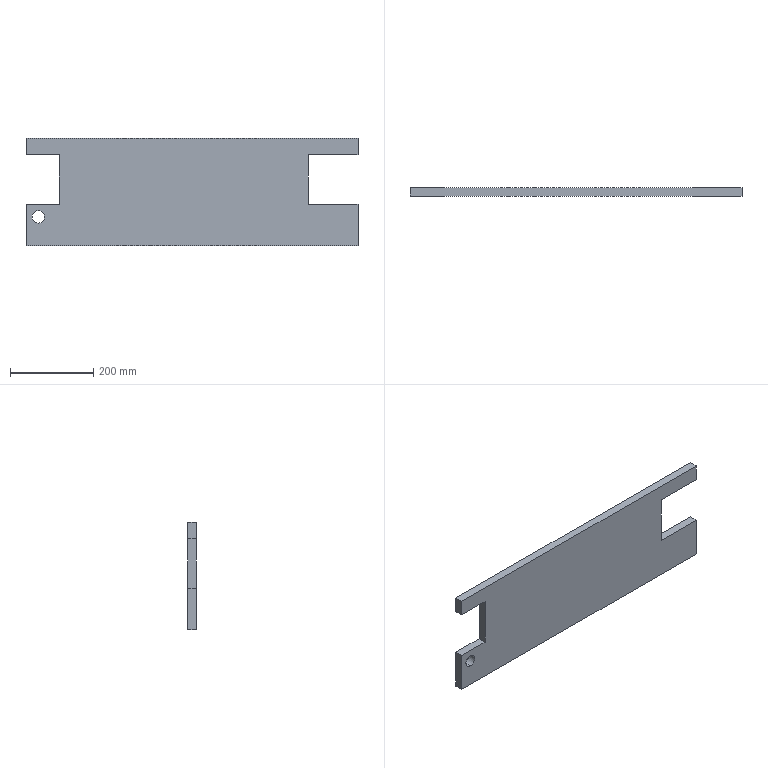Component | SolidWorks | JF21-80.1-1-3(_)-1-SOLID51-1 | 1 solid | 16 faces | box 800 x 20 x 260 mm | volume 3665863 mm3 | plane 14 | cylinder 2 | commonest cylinder face diameters 30 x2
STEP:
#1=CARTESIAN_POINT('',(-14.567,-32.283,43.11));
#2=VERTEX_POINT('',#1);
#3=CARTESIAN_POINT('',(-14.567,-32.283,44.291));
#4=VERTEX_POINT('',#3);
#5=CARTESIAN_POINT('',(-14.567,-32.283,43.701));
#6=DIRECTION('',(0.,1.,0.));
#7=DIRECTION('',(0.,0.,1.));
#8=AXIS2_PLACEMENT_3D('',#5,#6,#7);
#9=CIRCLE('',#8,0.5906);
#10=EDGE_CURVE('',#2,#4,#9,.T.);
#11=ORIENTED_EDGE('',*,*,#10,.F.);
#12=CARTESIAN_POINT('',(-14.567,-31.496,43.11));
#13=VERTEX_POINT('',#12);
#14=CARTESIAN_POINT('',(-14.567,-32.283,43.11));
#15=DIRECTION('',(0.,1.,0.));
#16=VECTOR('',#15,39.37);
#17=LINE('',#14,#16);
#18=EDGE_CURVE('',#2,#13,#17,.T.);
#19=ORIENTED_EDGE('',*,*,#18,.T.);
#20=CARTESIAN_POINT('',(-14.567,-31.496,44.291));
#21=VERTEX_POINT('',#20);
#22=CARTESIAN_POINT('',(-14.567,-31.496,43.701));
#23=DIRECTION('',(0.,1.,0.));
#24=DIRECTION('',(0.,0.,1.));
#25=AXIS2_PLACEMENT_3D('',#22,#23,#24);
#26=CIRCLE('',#25,0.5906);
#27=EDGE_CURVE('',#13,#21,#26,.T.);
#28=ORIENTED_EDGE('',*,*,#27,.T.);
#29=CARTESIAN_POINT('',(-14.567,-32.283,44.291));
#30=DIRECTION('',(0.,1.,0.));
#31=VECTOR('',#30,39.37);
#32=LINE('',#29,#31);
#33=EDGE_CURVE('',#4,#21,#32,.T.);
#34=ORIENTED_EDGE('',*,*,#33,.F.);
#35=EDGE_LOOP('',(#11,#19,#28,#34));
#36=FACE_OUTER_BOUND('',#35,.T.);
#37=CARTESIAN_POINT('',(-14.567,-32.283,43.701));
#38=DIRECTION('',(0.,1.,0.));
#39=DIRECTION('',(0.,0.,-1.));
#40=AXIS2_PLACEMENT_3D('',#37,#38,#39);
#41=CYLINDRICAL_SURFACE('',#40,0.5906);
#42=ADVANCED_FACE('',(#36),#41,.F.);
#43=CARTESIAN_POINT('',(15.748,-31.496,51.181));
#44=VERTEX_POINT('',#43);
#45=CARTESIAN_POINT('',(15.748,-31.496,49.606));
#46=VERTEX_POINT('',#45);
#47=CARTESIAN_POINT('',(15.748,-31.496,51.181));
#48=DIRECTION('',(0.,0.,-1.));
#49=VECTOR('',#48,39.37);
#50=LINE('',#47,#49);
#51=EDGE_CURVE('',#44,#46,#50,.T.);
#52=ORIENTED_EDGE('',*,*,#51,.F.);
#53=CARTESIAN_POINT('',(15.748,-32.283,51.181));
#54=VERTEX_POINT('',#53);
#55=CARTESIAN_POINT('',(15.748,-32.283,51.181));
#56=DIRECTION('',(0.,1.,0.));
#57=VECTOR('',#56,39.37);
#58=LINE('',#55,#57);
#59=EDGE_CURVE('',#54,#44,#58,.T.);
#60=ORIENTED_EDGE('',*,*,#59,.F.);
#61=CARTESIAN_POINT('',(15.748,-32.283,49.606));
#62=VERTEX_POINT('',#61);
#63=CARTESIAN_POINT('',(15.748,-32.283,51.181));
#64=DIRECTION('',(0.,0.,-1.));
#65=VECTOR('',#64,39.37);
#66=LINE('',#63,#65);
#67=EDGE_CURVE('',#54,#62,#66,.T.);
#68=ORIENTED_EDGE('',*,*,#67,.T.);
#69=CARTESIAN_POINT('',(15.748,-32.283,49.606));
#70=DIRECTION('',(0.,1.,0.));
#71=VECTOR('',#70,39.37);
#72=LINE('',#69,#71);
#73=EDGE_CURVE('',#62,#46,#72,.T.);
#74=ORIENTED_EDGE('',*,*,#73,.T.);
#75=EDGE_LOOP('',(#52,#60,#68,#74));
#76=FACE_OUTER_BOUND('',#75,.T.);
#77=CARTESIAN_POINT('',(15.748,-32.283,51.181));
#78=DIRECTION('',(1.,0.,0.));
#79=DIRECTION('',(0.,0.,1.));
#80=AXIS2_PLACEMENT_3D('',#77,#78,#79);
#81=PLANE('',#80);
#82=ADVANCED_FACE('',(#76),#81,.T.);
#83=CARTESIAN_POINT('',(-15.748,-31.496,51.181));
#84=VERTEX_POINT('',#83);
#85=CARTESIAN_POINT('',(15.748,-31.496,51.181));
#86=DIRECTION('',(1.,0.,0.));
#87=VECTOR('',#86,39.37);
#88=LINE('',#85,#87);
#89=EDGE_CURVE('',#84,#44,#88,.T.);
#90=ORIENTED_EDGE('',*,*,#89,.F.);
#91=CARTESIAN_POINT('',(-15.748,-32.283,51.181));
#92=VERTEX_POINT('',#91);
#93=CARTESIAN_POINT('',(-15.748,-32.283,51.181));
#94=DIRECTION('',(0.,1.,0.));
#95=VECTOR('',#94,39.37);
#96=LINE('',#93,#95);
#97=EDGE_CURVE('',#92,#84,#96,.T.);
#98=ORIENTED_EDGE('',*,*,#97,.F.);
#99=CARTESIAN_POINT('',(15.748,-32.283,51.181));
#100=DIRECTION('',(1.,0.,0.));
#101=VECTOR('',#100,39.37);
#102=LINE('',#99,#101);
#103=EDGE_CURVE('',#92,#54,#102,.T.);
#104=ORIENTED_EDGE('',*,*,#103,.T.);
#105=ORIENTED_EDGE('',*,*,#59,.T.);
#106=EDGE_LOOP('',(#90,#98,#104,#105));
#107=FACE_OUTER_BOUND('',#106,.T.);
#108=CARTESIAN_POINT('',(15.748,-32.283,51.181));
#109=DIRECTION('',(0.,0.,1.));
#110=DIRECTION('',(-1.,0.,0.));
#111=AXIS2_PLACEMENT_3D('',#108,#109,#110);
#112=PLANE('',#111);
#113=ADVANCED_FACE('',(#107),#112,.T.);
#114=CARTESIAN_POINT('',(-15.748,-31.496,49.606));
#115=VERTEX_POINT('',#114);
#116=CARTESIAN_POINT('',(-15.748,-31.496,51.181));
#117=DIRECTION('',(0.,0.,1.));
#118=VECTOR('',#117,39.37);
#119=LINE('',#116,#118);
#120=EDGE_CURVE('',#115,#84,#119,.T.);
#121=ORIENTED_EDGE('',*,*,#120,.F.);
#122=CARTESIAN_POINT('',(-15.748,-32.283,49.606));
#123=VERTEX_POINT('',#122);
#124=CARTESIAN_POINT('',(-15.748,-32.283,49.606));
#125=DIRECTION('',(0.,1.,0.));
#126=VECTOR('',#125,39.37);
#127=LINE('',#124,#126);
#128=EDGE_CURVE('',#123,#115,#127,.T.);
#129=ORIENTED_EDGE('',*,*,#128,.F.);
#130=CARTESIAN_POINT('',(-15.748,-32.283,51.181));
#131=DIRECTION('',(0.,0.,1.));
#132=VECTOR('',#131,39.37);
#133=LINE('',#130,#132);
#134=EDGE_CURVE('',#123,#92,#133,.T.);
#135=ORIENTED_EDGE('',*,*,#134,.T.);
#136=ORIENTED_EDGE('',*,*,#97,.T.);
#137=EDGE_LOOP('',(#121,#129,#135,#136));
#138=FACE_OUTER_BOUND('',#137,.T.);
#139=CARTESIAN_POINT('',(-15.748,-32.283,51.181));
#140=DIRECTION('',(-1.,0.,0.));
#141=DIRECTION('',(0.,0.,-1.));
#142=AXIS2_PLACEMENT_3D('',#139,#140,#141);
#143=PLANE('',#142);
#144=ADVANCED_FACE('',(#138),#143,.T.);
#145=CARTESIAN_POINT('',(-12.598,-31.496,49.606));
#146=VERTEX_POINT('',#145);
#147=CARTESIAN_POINT('',(-12.598,-31.496,49.606));
#148=DIRECTION('',(-1.,0.,0.));
#149=VECTOR('',#148,39.37);
#150=LINE('',#147,#149);
#151=EDGE_CURVE('',#146,#115,#150,.T.);
#152=ORIENTED_EDGE('',*,*,#151,.F.);
#153=CARTESIAN_POINT('',(-12.598,-32.283,49.606));
#154=VERTEX_POINT('',#153);
#155=CARTESIAN_POINT('',(-12.598,-32.283,49.606));
#156=DIRECTION('',(0.,1.,0.));
#157=VECTOR('',#156,39.37);
#158=LINE('',#155,#157);
#159=EDGE_CURVE('',#154,#146,#158,.T.);
#160=ORIENTED_EDGE('',*,*,#159,.F.);
#161=CARTESIAN_POINT('',(-12.598,-32.283,49.606));
#162=DIRECTION('',(-1.,0.,0.));
#163=VECTOR('',#162,39.37);
#164=LINE('',#161,#163);
#165=EDGE_CURVE('',#154,#123,#164,.T.);
#166=ORIENTED_EDGE('',*,*,#165,.T.);
#167=ORIENTED_EDGE('',*,*,#128,.T.);
#168=EDGE_LOOP('',(#152,#160,#166,#167));
#169=FACE_OUTER_BOUND('',#168,.T.);
#170=CARTESIAN_POINT('',(-12.598,-32.283,49.606));
#171=DIRECTION('',(0.,0.,-1.));
#172=DIRECTION('',(1.,0.,0.));
#173=AXIS2_PLACEMENT_3D('',#170,#171,#172);
#174=PLANE('',#173);
#175=ADVANCED_FACE('',(#169),#174,.T.);
#176=CARTESIAN_POINT('',(-12.598,-31.496,44.882));
#177=VERTEX_POINT('',#176);
#178=CARTESIAN_POINT('',(-12.598,-31.496,49.606));
#179=DIRECTION('',(0.,0.,1.));
#180=VECTOR('',#179,39.37);
#181=LINE('',#178,#180);
#182=EDGE_CURVE('',#177,#146,#181,.T.);
#183=ORIENTED_EDGE('',*,*,#182,.F.);
#184=CARTESIAN_POINT('',(-12.598,-32.283,44.882));
#185=VERTEX_POINT('',#184);
#186=CARTESIAN_POINT('',(-12.598,-32.283,44.882));
#187=DIRECTION('',(0.,1.,0.));
#188=VECTOR('',#187,39.37);
#189=LINE('',#186,#188);
#190=EDGE_CURVE('',#185,#177,#189,.T.);
#191=ORIENTED_EDGE('',*,*,#190,.F.);
#192=CARTESIAN_POINT('',(-12.598,-32.283,49.606));
#193=DIRECTION('',(0.,0.,1.));
#194=VECTOR('',#193,39.37);
#195=LINE('',#192,#194);
#196=EDGE_CURVE('',#185,#154,#195,.T.);
#197=ORIENTED_EDGE('',*,*,#196,.T.);
#198=ORIENTED_EDGE('',*,*,#159,.T.);
#199=EDGE_LOOP('',(#183,#191,#197,#198));
#200=FACE_OUTER_BOUND('',#199,.T.);
#201=CARTESIAN_POINT('',(-12.598,-32.283,49.606));
#202=DIRECTION('',(-1.,0.,0.));
#203=DIRECTION('',(-0.,0.,-1.));
#204=AXIS2_PLACEMENT_3D('',#201,#202,#203);
#205=PLANE('',#204);
#206=ADVANCED_FACE('',(#200),#205,.T.);
#207=CARTESIAN_POINT('',(-15.748,-31.496,44.882));
#208=VERTEX_POINT('',#207);
#209=CARTESIAN_POINT('',(-15.748,-31.496,44.882));
#210=DIRECTION('',(1.,0.,0.));
#211=VECTOR('',#210,39.37);
#212=LINE('',#209,#211);
#213=EDGE_CURVE('',#208,#177,#212,.T.);
#214=ORIENTED_EDGE('',*,*,#213,.F.);
#215=CARTESIAN_POINT('',(-15.748,-32.283,44.882));
#216=VERTEX_POINT('',#215);
#217=CARTESIAN_POINT('',(-15.748,-32.283,44.882));
#218=DIRECTION('',(0.,1.,0.));
#219=VECTOR('',#218,39.37);
#220=LINE('',#217,#219);
#221=EDGE_CURVE('',#216,#208,#220,.T.);
#222=ORIENTED_EDGE('',*,*,#221,.F.);
#223=CARTESIAN_POINT('',(-15.748,-32.283,44.882));
#224=DIRECTION('',(1.,0.,0.));
#225=VECTOR('',#224,39.37);
#226=LINE('',#223,#225);
#227=EDGE_CURVE('',#216,#185,#226,.T.);
#228=ORIENTED_EDGE('',*,*,#227,.T.);
#229=ORIENTED_EDGE('',*,*,#190,.T.);
#230=EDGE_LOOP('',(#214,#222,#228,#229));
#231=FACE_OUTER_BOUND('',#230,.T.);
#232=CARTESIAN_POINT('',(-15.748,-32.283,44.882));
#233=DIRECTION('',(0.,0.,1.));
#234=DIRECTION('',(-1.,0.,0.));
#235=AXIS2_PLACEMENT_3D('',#232,#233,#234);
#236=PLANE('',#235);
#237=ADVANCED_FACE('',(#231),#236,.T.);
#238=CARTESIAN_POINT('',(-15.748,-31.496,40.945));
#239=VERTEX_POINT('',#238);
#240=CARTESIAN_POINT('',(-15.748,-31.496,44.882));
#241=DIRECTION('',(0.,0.,1.));
#242=VECTOR('',#241,39.37);
#243=LINE('',#240,#242);
#244=EDGE_CURVE('',#239,#208,#243,.T.);
#245=ORIENTED_EDGE('',*,*,#244,.F.);
#246=CARTESIAN_POINT('',(-15.748,-32.283,40.945));
#247=VERTEX_POINT('',#246);
#248=CARTESIAN_POINT('',(-15.748,-32.283,40.945));
#249=DIRECTION('',(0.,1.,0.));
#250=VECTOR('',#249,39.37);
#251=LINE('',#248,#250);
#252=EDGE_CURVE('',#247,#239,#251,.T.);
#253=ORIENTED_EDGE('',*,*,#252,.F.);
#254=CARTESIAN_POINT('',(-15.748,-32.283,44.882));
#255=DIRECTION('',(0.,0.,1.));
#256=VECTOR('',#255,39.37);
#257=LINE('',#254,#256);
#258=EDGE_CURVE('',#247,#216,#257,.T.);
#259=ORIENTED_EDGE('',*,*,#258,.T.);
#260=ORIENTED_EDGE('',*,*,#221,.T.);
#261=EDGE_LOOP('',(#245,#253,#259,#260));
#262=FACE_OUTER_BOUND('',#261,.T.);
#263=CARTESIAN_POINT('',(-15.748,-32.283,44.882));
#264=DIRECTION('',(-1.,0.,0.));
#265=DIRECTION('',(0.,0.,-1.));
#266=AXIS2_PLACEMENT_3D('',#263,#264,#265);
#267=PLANE('',#266);
#268=ADVANCED_FACE('',(#262),#267,.T.);
#269=CARTESIAN_POINT('',(15.748,-31.496,40.945));
#270=VERTEX_POINT('',#269);
#271=CARTESIAN_POINT('',(15.748,-31.496,40.945));
#272=DIRECTION('',(-1.,0.,0.));
#273=VECTOR('',#272,39.37);
#274=LINE('',#271,#273);
#275=EDGE_CURVE('',#270,#239,#274,.T.);
#276=ORIENTED_EDGE('',*,*,#275,.F.);
#277=CARTESIAN_POINT('',(15.748,-32.283,40.945));
#278=VERTEX_POINT('',#277);
#279=CARTESIAN_POINT('',(15.748,-32.283,40.945));
#280=DIRECTION('',(0.,1.,0.));
#281=VECTOR('',#280,39.37);
#282=LINE('',#279,#281);
#283=EDGE_CURVE('',#278,#270,#282,.T.);
#284=ORIENTED_EDGE('',*,*,#283,.F.);
#285=CARTESIAN_POINT('',(15.748,-32.283,40.945));
#286=DIRECTION('',(-1.,0.,0.));
#287=VECTOR('',#286,39.37);
#288=LINE('',#285,#287);
#289=EDGE_CURVE('',#278,#247,#288,.T.);
#290=ORIENTED_EDGE('',*,*,#289,.T.);
#291=ORIENTED_EDGE('',*,*,#252,.T.);
#292=EDGE_LOOP('',(#276,#284,#290,#291));
#293=FACE_OUTER_BOUND('',#292,.T.);
#294=CARTESIAN_POINT('',(15.748,-32.283,40.945));
#295=DIRECTION('',(0.,0.,-1.));
#296=DIRECTION('',(1.,0.,0.));
#297=AXIS2_PLACEMENT_3D('',#294,#295,#296);
#298=PLANE('',#297);
#299=ADVANCED_FACE('',(#293),#298,.T.);
#300=CARTESIAN_POINT('',(15.748,-31.496,44.882));
#301=VERTEX_POINT('',#300);
#302=CARTESIAN_POINT('',(15.748,-31.496,44.882));
#303=DIRECTION('',(-0.,0.,-1.));
#304=VECTOR('',#303,39.37);
#305=LINE('',#302,#304);
#306=EDGE_CURVE('',#301,#270,#305,.T.);
#307=ORIENTED_EDGE('',*,*,#306,.F.);
#308=CARTESIAN_POINT('',(15.748,-32.283,44.882));
#309=VERTEX_POINT('',#308);
#310=CARTESIAN_POINT('',(15.748,-32.283,44.882));
#311=DIRECTION('',(0.,1.,0.));
#312=VECTOR('',#311,39.37);
#313=LINE('',#310,#312);
#314=EDGE_CURVE('',#309,#301,#313,.T.);
#315=ORIENTED_EDGE('',*,*,#314,.F.);
#316=CARTESIAN_POINT('',(15.748,-32.283,44.882));
#317=DIRECTION('',(-0.,0.,-1.));
#318=VECTOR('',#317,39.37);
#319=LINE('',#316,#318);
#320=EDGE_CURVE('',#309,#278,#319,.T.);
#321=ORIENTED_EDGE('',*,*,#320,.T.);
#322=ORIENTED_EDGE('',*,*,#283,.T.);
#323=EDGE_LOOP('',(#307,#315,#321,#322));
#324=FACE_OUTER_BOUND('',#323,.T.);
#325=CARTESIAN_POINT('',(15.748,-32.283,44.882));
#326=DIRECTION('',(1.,0.,-0.));
#327=DIRECTION('',(0.,0.,1.));
#328=AXIS2_PLACEMENT_3D('',#325,#326,#327);
#329=PLANE('',#328);
#330=ADVANCED_FACE('',(#324),#329,.T.);
#331=CARTESIAN_POINT('',(11.024,-31.496,44.882));
#332=VERTEX_POINT('',#331);
#333=CARTESIAN_POINT('',(11.024,-31.496,44.882));
#334=DIRECTION('',(1.,0.,0.));
#335=VECTOR('',#334,39.37);
#336=LINE('',#333,#335);
#337=EDGE_CURVE('',#332,#301,#336,.T.);
#338=ORIENTED_EDGE('',*,*,#337,.F.);
#339=CARTESIAN_POINT('',(11.024,-32.283,44.882));
#340=VERTEX_POINT('',#339);
#341=CARTESIAN_POINT('',(11.024,-32.283,44.882));
#342=DIRECTION('',(0.,1.,0.));
#343=VECTOR('',#342,39.37);
#344=LINE('',#341,#343);
#345=EDGE_CURVE('',#340,#332,#344,.T.);
#346=ORIENTED_EDGE('',*,*,#345,.F.);
#347=CARTESIAN_POINT('',(11.024,-32.283,44.882));
#348=DIRECTION('',(1.,0.,0.));
#349=VECTOR('',#348,39.37);
#350=LINE('',#347,#349);
#351=EDGE_CURVE('',#340,#309,#350,.T.);
#352=ORIENTED_EDGE('',*,*,#351,.T.);
#353=ORIENTED_EDGE('',*,*,#314,.T.);
#354=EDGE_LOOP('',(#338,#346,#352,#353));
#355=FACE_OUTER_BOUND('',#354,.T.);
#356=CARTESIAN_POINT('',(11.024,-32.283,44.882));
#357=DIRECTION('',(0.,0.,1.));
#358=DIRECTION('',(-1.,0.,0.));
#359=AXIS2_PLACEMENT_3D('',#356,#357,#358);
#360=PLANE('',#359);
#361=ADVANCED_FACE('',(#355),#360,.T.);
#362=CARTESIAN_POINT('',(11.024,-31.496,49.606));
#363=VERTEX_POINT('',#362);
#364=CARTESIAN_POINT('',(11.024,-31.496,49.606));
#365=DIRECTION('',(0.,0.,-1.));
#366=VECTOR('',#365,39.37);
#367=LINE('',#364,#366);
#368=EDGE_CURVE('',#363,#332,#367,.T.);
#369=ORIENTED_EDGE('',*,*,#368,.F.);
#370=CARTESIAN_POINT('',(11.024,-32.283,49.606));
#371=VERTEX_POINT('',#370);
#372=CARTESIAN_POINT('',(11.024,-32.283,49.606));
#373=DIRECTION('',(0.,1.,0.));
#374=VECTOR('',#373,39.37);
#375=LINE('',#372,#374);
#376=EDGE_CURVE('',#371,#363,#375,.T.);
#377=ORIENTED_EDGE('',*,*,#376,.F.);
#378=CARTESIAN_POINT('',(11.024,-32.283,49.606));
#379=DIRECTION('',(0.,0.,-1.));
#380=VECTOR('',#379,39.37);
#381=LINE('',#378,#380);
#382=EDGE_CURVE('',#371,#340,#381,.T.);
#383=ORIENTED_EDGE('',*,*,#382,.T.);
#384=ORIENTED_EDGE('',*,*,#345,.T.);
#385=EDGE_LOOP('',(#369,#377,#383,#384));
#386=FACE_OUTER_BOUND('',#385,.T.);
#387=CARTESIAN_POINT('',(11.024,-32.283,49.606));
#388=DIRECTION('',(1.,0.,0.));
#389=DIRECTION('',(0.,0.,1.));
#390=AXIS2_PLACEMENT_3D('',#387,#388,#389);
#391=PLANE('',#390);
#392=ADVANCED_FACE('',(#386),#391,.T.);
#393=CARTESIAN_POINT('',(15.748,-31.496,49.606));
#394=DIRECTION('',(-1.,0.,0.));
#395=VECTOR('',#394,39.37);
#396=LINE('',#393,#395);
#397=EDGE_CURVE('',#46,#363,#396,.T.);
#398=ORIENTED_EDGE('',*,*,#397,.F.);
#399=ORIENTED_EDGE('',*,*,#73,.F.);
#400=CARTESIAN_POINT('',(15.748,-32.283,49.606));
#401=DIRECTION('',(-1.,0.,0.));
#402=VECTOR('',#401,39.37);
#403=LINE('',#400,#402);
#404=EDGE_CURVE('',#62,#371,#403,.T.);
#405=ORIENTED_EDGE('',*,*,#404,.T.);
#406=ORIENTED_EDGE('',*,*,#376,.T.);
#407=EDGE_LOOP('',(#398,#399,#405,#406));
#408=FACE_OUTER_BOUND('',#407,.T.);
#409=CARTESIAN_POINT('',(15.748,-32.283,49.606));
#410=DIRECTION('',(0.,0.,-1.));
#411=DIRECTION('',(1.,0.,0.));
#412=AXIS2_PLACEMENT_3D('',#409,#410,#411);
#413=PLANE('',#412);
#414=ADVANCED_FACE('',(#408),#413,.T.);
#415=CARTESIAN_POINT('',(-14.567,-32.283,43.701));
#416=DIRECTION('',(0.,1.,0.));
#417=DIRECTION('',(0.,0.,1.));
#418=AXIS2_PLACEMENT_3D('',#415,#416,#417);
#419=CIRCLE('',#418,0.5906);
#420=EDGE_CURVE('',#4,#2,#419,.T.);
#421=ORIENTED_EDGE('',*,*,#420,.T.);
#422=ORIENTED_EDGE('',*,*,#10,.T.);
#423=EDGE_LOOP('',(#421,#422));
#424=FACE_BOUND('',#423,.T.);
#425=ORIENTED_EDGE('',*,*,#67,.F.);
#426=ORIENTED_EDGE('',*,*,#103,.F.);
#427=ORIENTED_EDGE('',*,*,#134,.F.);
#428=ORIENTED_EDGE('',*,*,#165,.F.);
#429=ORIENTED_EDGE('',*,*,#196,.F.);
#430=ORIENTED_EDGE('',*,*,#227,.F.);
#431=ORIENTED_EDGE('',*,*,#258,.F.);
#432=ORIENTED_EDGE('',*,*,#289,.F.);
#433=ORIENTED_EDGE('',*,*,#320,.F.);
#434=ORIENTED_EDGE('',*,*,#351,.F.);
#435=ORIENTED_EDGE('',*,*,#382,.F.);
#436=ORIENTED_EDGE('',*,*,#404,.F.);
#437=EDGE_LOOP('',(#425,#426,#427,#428,#429,#430,#431,#432,#433,#434,#435,#436));
#438=FACE_OUTER_BOUND('',#437,.T.);
#439=CARTESIAN_POINT('',(15.748,-32.283,49.606));
#440=DIRECTION('',(0.,1.,0.));
#441=DIRECTION('',(0.,0.,-1.));
#442=AXIS2_PLACEMENT_3D('',#439,#440,#441);
#443=PLANE('',#442);
#444=ADVANCED_FACE('',(#424,#438),#443,.F.);
#445=CARTESIAN_POINT('',(-14.567,-31.496,43.701));
#446=DIRECTION('',(0.,1.,0.));
#447=DIRECTION('',(0.,0.,1.));
#448=AXIS2_PLACEMENT_3D('',#445,#446,#447);
#449=CIRCLE('',#448,0.5906);
#450=EDGE_CURVE('',#21,#13,#449,.T.);
#451=ORIENTED_EDGE('',*,*,#450,.F.);
#452=ORIENTED_EDGE('',*,*,#27,.F.);
#453=EDGE_LOOP('',(#451,#452));
#454=FACE_BOUND('',#453,.T.);
#455=ORIENTED_EDGE('',*,*,#51,.T.);
#456=ORIENTED_EDGE('',*,*,#397,.T.);
#457=ORIENTED_EDGE('',*,*,#368,.T.);
#458=ORIENTED_EDGE('',*,*,#337,.T.);
#459=ORIENTED_EDGE('',*,*,#306,.T.);
#460=ORIENTED_EDGE('',*,*,#275,.T.);
#461=ORIENTED_EDGE('',*,*,#244,.T.);
#462=ORIENTED_EDGE('',*,*,#213,.T.);
#463=ORIENTED_EDGE('',*,*,#182,.T.);
#464=ORIENTED_EDGE('',*,*,#151,.T.);
#465=ORIENTED_EDGE('',*,*,#120,.T.);
#466=ORIENTED_EDGE('',*,*,#89,.T.);
#467=EDGE_LOOP('',(#455,#456,#457,#458,#459,#460,#461,#462,#463,#464,#465,#466));
#468=FACE_OUTER_BOUND('',#467,.T.);
#469=CARTESIAN_POINT('',(15.748,-31.496,49.606));
#470=DIRECTION('',(0.,1.,0.));
#471=DIRECTION('',(0.,0.,-1.));
#472=AXIS2_PLACEMENT_3D('',#469,#470,#471);
#473=PLANE('',#472);
#474=ADVANCED_FACE('',(#454,#468),#473,.T.);
#475=ORIENTED_EDGE('',*,*,#18,.F.);
#476=ORIENTED_EDGE('',*,*,#420,.F.);
#477=ORIENTED_EDGE('',*,*,#33,.T.);
#478=ORIENTED_EDGE('',*,*,#450,.T.);
#479=EDGE_LOOP('',(#475,#476,#477,#478));
#480=FACE_OUTER_BOUND('',#479,.T.);
#481=CARTESIAN_POINT('',(-14.567,-32.283,43.701));
#482=DIRECTION('',(0.,1.,0.));
#483=DIRECTION('',(0.,0.,-1.));
#484=AXIS2_PLACEMENT_3D('',#481,#482,#483);
#485=CYLINDRICAL_SURFACE('',#484,0.5906);
#486=ADVANCED_FACE('',(#480),#485,.F.);
#487=CLOSED_SHELL('',(#42,#82,#113,#144,#175,#206,#237,#268,#299,#330,#361,#392,#414,#444,#474,#486));
#488=MANIFOLD_SOLID_BREP('',#487);
#489=CARTESIAN_POINT('',(0.,0.,0.));
#490=DIRECTION('',(0.,0.,1.));
#491=DIRECTION('',(1.,0.,0.));
#492=AXIS2_PLACEMENT_3D('',#489,#490,#491);
#493=(LENGTH_UNIT()NAMED_UNIT(*)SI_UNIT($,.METRE.));
#494=LENGTH_MEASURE_WITH_UNIT(LENGTH_MEASURE(0.0254),#493);
#495=DIMENSIONAL_EXPONENTS(1.,0.,0.,0.,0.,0.,0.);
#496=(CONVERSION_BASED_UNIT('',#494)LENGTH_UNIT()NAMED_UNIT(#495));
#497=UNCERTAINTY_MEASURE_WITH_UNIT(LENGTH_MEASURE(0.00001),#496,'','');
#498=(NAMED_UNIT(*)PLANE_ANGLE_UNIT()SI_UNIT($,.RADIAN.));
#499=(NAMED_UNIT(*)SI_UNIT($,.STERADIAN.)SOLID_ANGLE_UNIT());
#500=(GEOMETRIC_REPRESENTATION_CONTEXT(3)GLOBAL_UNCERTAINTY_ASSIGNED_CONTEXT((#497))GLOBAL_UNIT_ASSIGNED_CONTEXT((#496,#498,#499))REPRESENTATION_CONTEXT('',''));
#501=ADVANCED_BREP_SHAPE_REPRESENTATION('',(#488,#492),#500);
#502=COLOUR_RGB('',0.7922,0.8196,0.9333);
#503=FILL_AREA_STYLE_COLOUR('',#502);
#504=FILL_AREA_STYLE('',(#503));
#505=SURFACE_STYLE_FILL_AREA(#504);
#506=SURFACE_SIDE_STYLE('',(#505));
#507=SURFACE_STYLE_USAGE(.BOTH.,#506);
#508=PRESENTATION_STYLE_ASSIGNMENT((#507));
#509=STYLED_ITEM('',(#508),#488);
#510=(LENGTH_UNIT()NAMED_UNIT(*)SI_UNIT($,.METRE.));
#511=LENGTH_MEASURE_WITH_UNIT(LENGTH_MEASURE(0.0254),#510);
#512=DIMENSIONAL_EXPONENTS(1.,0.,0.,0.,0.,0.,0.);
#513=(CONVERSION_BASED_UNIT('',#511)LENGTH_UNIT()NAMED_UNIT(#512));
#514=UNCERTAINTY_MEASURE_WITH_UNIT(LENGTH_MEASURE(0.00001),#513,'','');
#515=(NAMED_UNIT(*)PLANE_ANGLE_UNIT()SI_UNIT($,.RADIAN.));
#516=(NAMED_UNIT(*)SI_UNIT($,.STERADIAN.)SOLID_ANGLE_UNIT());
#517=(GEOMETRIC_REPRESENTATION_CONTEXT(3)GLOBAL_UNCERTAINTY_ASSIGNED_CONTEXT((#514))GLOBAL_UNIT_ASSIGNED_CONTEXT((#513,#515,#516))REPRESENTATION_CONTEXT('',''));
#518=MECHANICAL_DESIGN_GEOMETRIC_PRESENTATION_REPRESENTATION('',(#509),#517);
#519=PRESENTATION_LAYER_ASSIGNMENT('','',(#509));